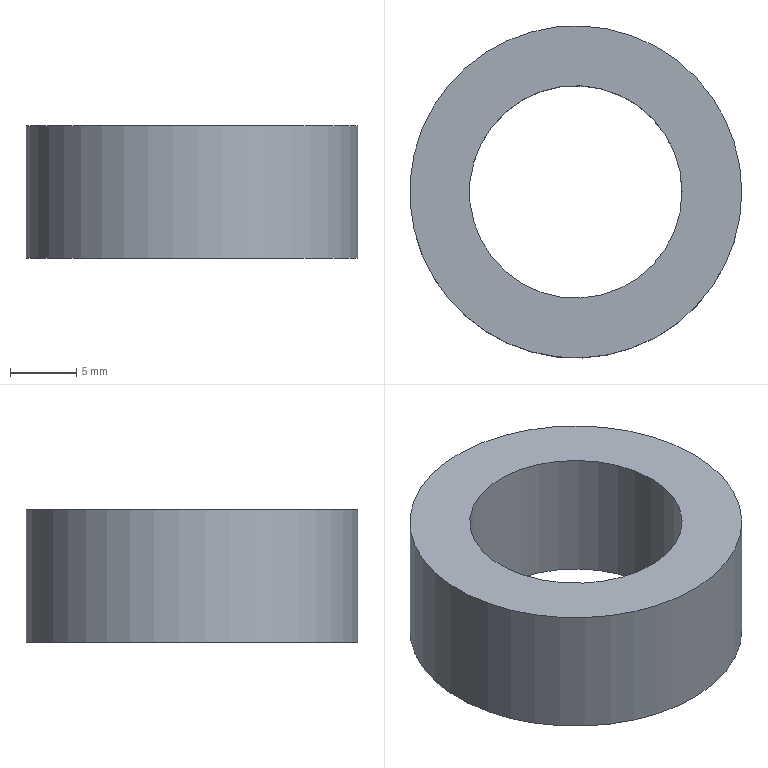Component | NX | PACKING | 1 solid | 4 faces | box 25 x 25 x 10 mm | volume 2898 mm3 | cylinder 2 | plane 2 | commonest cylinder face diameters 25 x1 16 x1
STEP:
#1=CARTESIAN_POINT('',(0.,0.,0.));
#2=DIRECTION('',(0.,0.,1.));
#3=DIRECTION('',(1.,0.,0.));
#4=AXIS2_PLACEMENT_3D('',#1,#2,#3);
#5=CARTESIAN_POINT('',(189.665,26.5,74.));
#6=VERTEX_POINT('',#5);
#7=CARTESIAN_POINT('',(177.165,26.5,74.));
#8=DIRECTION('',(0.,0.,1.));
#9=DIRECTION('',(1.,0.,0.));
#10=AXIS2_PLACEMENT_3D('',#7,#8,#9);
#11=CIRCLE('',#10,12.5);
#12=CARTESIAN_POINT('',(177.165,26.5,74.));
#13=DIRECTION('',(0.,0.,-1.));
#14=DIRECTION('',(-1.,0.,0.));
#15=AXIS2_PLACEMENT_3D('',#12,#13,#14);
#16=CYLINDRICAL_SURFACE('',#15,12.5);
#17=CARTESIAN_POINT('',(9.425,0.));
#18=DIRECTION('',(-1.,0.));
#19=VECTOR('',#18,1.);
#20=LINE('',#17,#19);
#21=(GEOMETRIC_REPRESENTATION_CONTEXT(2)PARAMETRIC_REPRESENTATION_CONTEXT()REPRESENTATION_CONTEXT('',''));
#22=DEFINITIONAL_REPRESENTATION('',(#20),#21);
#23=PCURVE('',#16,#22);
#24=CARTESIAN_POINT('',(177.165,26.5,74.));
#25=DIRECTION('',(0.,0.,1.));
#26=DIRECTION('',(1.,0.,0.));
#27=AXIS2_PLACEMENT_3D('',#24,#25,#26);
#28=PLANE('',#27);
#29=CARTESIAN_POINT('',(0.,0.));
#30=DIRECTION('',(1.,0.));
#31=AXIS2_PLACEMENT_2D('',#29,#30);
#32=CIRCLE('',#31,12.5);
#33=(GEOMETRIC_REPRESENTATION_CONTEXT(2)PARAMETRIC_REPRESENTATION_CONTEXT()REPRESENTATION_CONTEXT('',''));
#34=DEFINITIONAL_REPRESENTATION('',(#32),#33);
#35=PCURVE('',#28,#34);
#36=SURFACE_CURVE('',#11,(#23,#35),.PCURVE_S1.);
#37=EDGE_CURVE('',#6,#6,#36,.T.);
#38=ORIENTED_EDGE('',*,*,#37,.F.);
#39=CARTESIAN_POINT('',(189.665,26.5,64.));
#40=VERTEX_POINT('',#39);
#41=CARTESIAN_POINT('',(189.665,26.5,74.));
#42=CARTESIAN_POINT('',(189.665,26.5,64.));
#43=B_SPLINE_CURVE_WITH_KNOTS('',1,(#41,#42),.UNSPECIFIED.,.F.,.F.,(2,2),(0.,10.),.PIECEWISE_BEZIER_KNOTS.);
#44=CARTESIAN_POINT('',(9.425,0.));
#45=DIRECTION('',(0.,1.));
#46=VECTOR('',#45,1.);
#47=LINE('',#44,#46);
#48=(GEOMETRIC_REPRESENTATION_CONTEXT(2)PARAMETRIC_REPRESENTATION_CONTEXT()REPRESENTATION_CONTEXT('',''));
#49=DEFINITIONAL_REPRESENTATION('',(#47),#48);
#50=PCURVE('',#16,#49);
#51=CARTESIAN_POINT('',(3.142,0.));
#52=DIRECTION('',(0.,1.));
#53=VECTOR('',#52,1.);
#54=LINE('',#51,#53);
#55=(GEOMETRIC_REPRESENTATION_CONTEXT(2)PARAMETRIC_REPRESENTATION_CONTEXT()REPRESENTATION_CONTEXT('',''));
#56=DEFINITIONAL_REPRESENTATION('',(#54),#55);
#57=PCURVE('',#16,#56);
#58=SEAM_CURVE('',#43,(#50,#57),.PCURVE_S1.);
#59=EDGE_CURVE('',#6,#40,#58,.T.);
#60=ORIENTED_EDGE('',*,*,#59,.T.);
#61=CARTESIAN_POINT('',(177.165,26.5,64.));
#62=DIRECTION('',(0.,0.,1.));
#63=DIRECTION('',(1.,0.,0.));
#64=AXIS2_PLACEMENT_3D('',#61,#62,#63);
#65=CIRCLE('',#64,12.5);
#66=CARTESIAN_POINT('',(9.425,10.));
#67=DIRECTION('',(-1.,0.));
#68=VECTOR('',#67,1.);
#69=LINE('',#66,#68);
#70=(GEOMETRIC_REPRESENTATION_CONTEXT(2)PARAMETRIC_REPRESENTATION_CONTEXT()REPRESENTATION_CONTEXT('',''));
#71=DEFINITIONAL_REPRESENTATION('',(#69),#70);
#72=PCURVE('',#16,#71);
#73=CARTESIAN_POINT('',(177.165,26.5,64.));
#74=DIRECTION('',(0.,0.,1.));
#75=DIRECTION('',(1.,0.,0.));
#76=AXIS2_PLACEMENT_3D('',#73,#74,#75);
#77=PLANE('',#76);
#78=CARTESIAN_POINT('',(0.,0.));
#79=DIRECTION('',(1.,0.));
#80=AXIS2_PLACEMENT_2D('',#78,#79);
#81=CIRCLE('',#80,12.5);
#82=(GEOMETRIC_REPRESENTATION_CONTEXT(2)PARAMETRIC_REPRESENTATION_CONTEXT()REPRESENTATION_CONTEXT('',''));
#83=DEFINITIONAL_REPRESENTATION('',(#81),#82);
#84=PCURVE('',#77,#83);
#85=SURFACE_CURVE('',#65,(#72,#84),.PCURVE_S1.);
#86=EDGE_CURVE('',#40,#40,#85,.T.);
#87=ORIENTED_EDGE('',*,*,#86,.T.);
#88=ORIENTED_EDGE('',*,*,#59,.F.);
#89=EDGE_LOOP('',(#38,#60,#87,#88));
#90=FACE_BOUND('',#89,.T.);
#91=ADVANCED_FACE('',(#90),#16,.T.);
#92=CARTESIAN_POINT('',(185.165,26.5,74.));
#93=VERTEX_POINT('',#92);
#94=CARTESIAN_POINT('',(177.165,26.5,74.));
#95=DIRECTION('',(0.,0.,1.));
#96=DIRECTION('',(1.,0.,0.));
#97=AXIS2_PLACEMENT_3D('',#94,#95,#96);
#98=CIRCLE('',#97,8.);
#99=CARTESIAN_POINT('',(177.165,26.5,74.));
#100=DIRECTION('',(0.,0.,-1.));
#101=DIRECTION('',(-1.,0.,0.));
#102=AXIS2_PLACEMENT_3D('',#99,#100,#101);
#103=CYLINDRICAL_SURFACE('',#102,8.);
#104=CARTESIAN_POINT('',(9.425,0.));
#105=DIRECTION('',(-1.,0.));
#106=VECTOR('',#105,1.);
#107=LINE('',#104,#106);
#108=(GEOMETRIC_REPRESENTATION_CONTEXT(2)PARAMETRIC_REPRESENTATION_CONTEXT()REPRESENTATION_CONTEXT('',''));
#109=DEFINITIONAL_REPRESENTATION('',(#107),#108);
#110=PCURVE('',#103,#109);
#111=CARTESIAN_POINT('',(0.,0.));
#112=DIRECTION('',(1.,0.));
#113=AXIS2_PLACEMENT_2D('',#111,#112);
#114=CIRCLE('',#113,8.);
#115=(GEOMETRIC_REPRESENTATION_CONTEXT(2)PARAMETRIC_REPRESENTATION_CONTEXT()REPRESENTATION_CONTEXT('',''));
#116=DEFINITIONAL_REPRESENTATION('',(#114),#115);
#117=PCURVE('',#28,#116);
#118=SURFACE_CURVE('',#98,(#110,#117),.PCURVE_S1.);
#119=EDGE_CURVE('',#93,#93,#118,.T.);
#120=ORIENTED_EDGE('',*,*,#119,.F.);
#121=CARTESIAN_POINT('',(185.165,26.5,64.));
#122=VERTEX_POINT('',#121);
#123=CARTESIAN_POINT('',(185.165,26.5,74.));
#124=CARTESIAN_POINT('',(185.165,26.5,64.));
#125=B_SPLINE_CURVE_WITH_KNOTS('',1,(#123,#124),.UNSPECIFIED.,.F.,.F.,(2,2),(0.,10.),.PIECEWISE_BEZIER_KNOTS.);
#126=CARTESIAN_POINT('',(9.425,0.));
#127=DIRECTION('',(0.,1.));
#128=VECTOR('',#127,1.);
#129=LINE('',#126,#128);
#130=(GEOMETRIC_REPRESENTATION_CONTEXT(2)PARAMETRIC_REPRESENTATION_CONTEXT()REPRESENTATION_CONTEXT('',''));
#131=DEFINITIONAL_REPRESENTATION('',(#129),#130);
#132=PCURVE('',#103,#131);
#133=CARTESIAN_POINT('',(3.142,0.));
#134=DIRECTION('',(0.,1.));
#135=VECTOR('',#134,1.);
#136=LINE('',#133,#135);
#137=(GEOMETRIC_REPRESENTATION_CONTEXT(2)PARAMETRIC_REPRESENTATION_CONTEXT()REPRESENTATION_CONTEXT('',''));
#138=DEFINITIONAL_REPRESENTATION('',(#136),#137);
#139=PCURVE('',#103,#138);
#140=SEAM_CURVE('',#125,(#132,#139),.PCURVE_S1.);
#141=EDGE_CURVE('',#93,#122,#140,.T.);
#142=ORIENTED_EDGE('',*,*,#141,.T.);
#143=CARTESIAN_POINT('',(177.165,26.5,64.));
#144=DIRECTION('',(0.,0.,1.));
#145=DIRECTION('',(1.,0.,0.));
#146=AXIS2_PLACEMENT_3D('',#143,#144,#145);
#147=CIRCLE('',#146,8.);
#148=CARTESIAN_POINT('',(9.425,10.));
#149=DIRECTION('',(-1.,0.));
#150=VECTOR('',#149,1.);
#151=LINE('',#148,#150);
#152=(GEOMETRIC_REPRESENTATION_CONTEXT(2)PARAMETRIC_REPRESENTATION_CONTEXT()REPRESENTATION_CONTEXT('',''));
#153=DEFINITIONAL_REPRESENTATION('',(#151),#152);
#154=PCURVE('',#103,#153);
#155=CARTESIAN_POINT('',(0.,0.));
#156=DIRECTION('',(1.,0.));
#157=AXIS2_PLACEMENT_2D('',#155,#156);
#158=CIRCLE('',#157,8.);
#159=(GEOMETRIC_REPRESENTATION_CONTEXT(2)PARAMETRIC_REPRESENTATION_CONTEXT()REPRESENTATION_CONTEXT('',''));
#160=DEFINITIONAL_REPRESENTATION('',(#158),#159);
#161=PCURVE('',#77,#160);
#162=SURFACE_CURVE('',#147,(#154,#161),.PCURVE_S1.);
#163=EDGE_CURVE('',#122,#122,#162,.T.);
#164=ORIENTED_EDGE('',*,*,#163,.T.);
#165=ORIENTED_EDGE('',*,*,#141,.F.);
#166=EDGE_LOOP('',(#120,#142,#164,#165));
#167=FACE_BOUND('',#166,.F.);
#168=ADVANCED_FACE('',(#167),#103,.F.);
#169=ORIENTED_EDGE('',*,*,#37,.T.);
#170=EDGE_LOOP('',(#169));
#171=FACE_BOUND('',#170,.T.);
#172=ORIENTED_EDGE('',*,*,#119,.F.);
#173=EDGE_LOOP('',(#172));
#174=FACE_BOUND('',#173,.T.);
#175=ADVANCED_FACE('',(#171,#174),#28,.T.);
#176=ORIENTED_EDGE('',*,*,#86,.F.);
#177=EDGE_LOOP('',(#176));
#178=FACE_BOUND('',#177,.T.);
#179=ORIENTED_EDGE('',*,*,#163,.T.);
#180=EDGE_LOOP('',(#179));
#181=FACE_BOUND('',#180,.T.);
#182=ADVANCED_FACE('',(#178,#181),#77,.F.);
#183=CLOSED_SHELL('',(#91,#168,#175,#182));
#184=MANIFOLD_SOLID_BREP('',#183);
#185=(LENGTH_UNIT()NAMED_UNIT(*)SI_UNIT(.MILLI.,.METRE.));
#186=UNCERTAINTY_MEASURE_WITH_UNIT(LENGTH_MEASURE(0.00001),#185,'','');
#187=(NAMED_UNIT(*)PLANE_ANGLE_UNIT()SI_UNIT($,.RADIAN.));
#188=(NAMED_UNIT(*)SI_UNIT($,.STERADIAN.)SOLID_ANGLE_UNIT());
#189=(GEOMETRIC_REPRESENTATION_CONTEXT(3)GLOBAL_UNCERTAINTY_ASSIGNED_CONTEXT((#186))GLOBAL_UNIT_ASSIGNED_CONTEXT((#185,#187,#188))REPRESENTATION_CONTEXT('',''));
#190=ADVANCED_BREP_SHAPE_REPRESENTATION('',(#4,#184),#189);